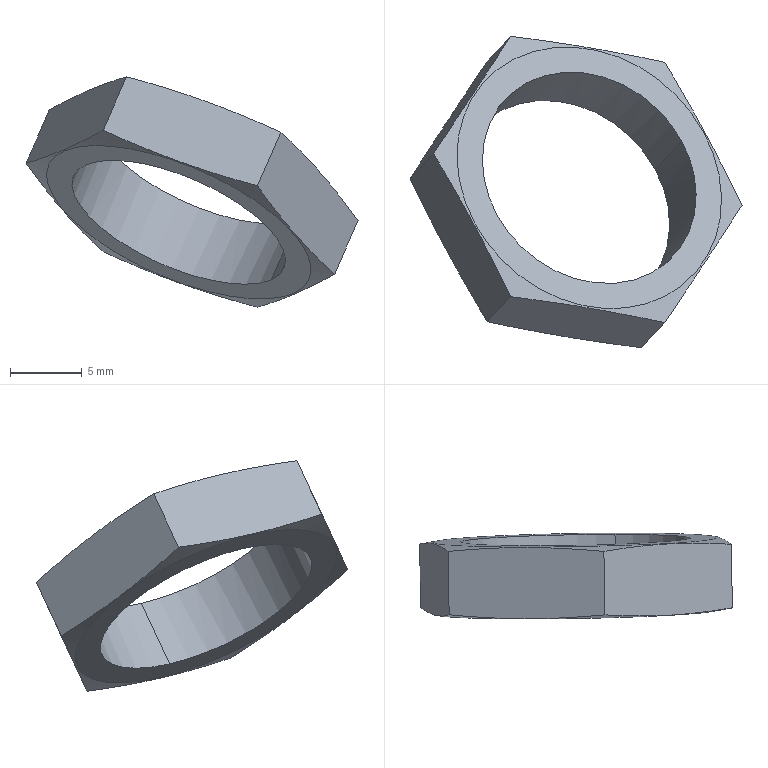Component | SolidWorks | 1369126_DSM_40_270_CC_HD_A_B_0-1_Flachmutter_M16x1_5_20-1 | 1 solid | 14 faces | box 23.1 x 21.66 x 16.04 mm | volume 720 mm3 | plane 8 | cone 4 | cylinder 2 | commonest cylinder face diameters 16 x2
STEP:
#1=COLOUR_RGB('',0.7922,0.8196,0.9333);
#2=FILL_AREA_STYLE_COLOUR('',#1);
#3=FILL_AREA_STYLE('',(#2));
#4=SURFACE_STYLE_FILL_AREA(#3);
#5=SURFACE_SIDE_STYLE('',(#4));
#6=SURFACE_STYLE_USAGE(.BOTH.,#5);
#7=PRESENTATION_STYLE_ASSIGNMENT((#6));
#8=CARTESIAN_POINT('',(-8.237,80.701,9.666));
#9=VERTEX_POINT('',#8);
#10=CARTESIAN_POINT('',(-7.73,80.902,9.351));
#11=VERTEX_POINT('',#10);
#12=CARTESIAN_POINT('',(-8.237,80.701,9.666));
#13=CARTESIAN_POINT('',(-8.246,80.719,9.662));
#14=CARTESIAN_POINT('',(-8.254,80.738,9.657));
#15=CARTESIAN_POINT('',(-8.267,80.775,9.645));
#16=CARTESIAN_POINT('',(-8.271,80.794,9.638));
#17=CARTESIAN_POINT('',(-8.276,80.832,9.622));
#18=CARTESIAN_POINT('',(-8.277,80.851,9.614));
#19=CARTESIAN_POINT('',(-8.274,80.888,9.596));
#20=CARTESIAN_POINT('',(-8.271,80.906,9.586));
#21=CARTESIAN_POINT('',(-8.261,80.94,9.565));
#22=CARTESIAN_POINT('',(-8.254,80.957,9.555));
#23=CARTESIAN_POINT('',(-8.237,80.987,9.533));
#24=CARTESIAN_POINT('',(-8.227,81.001,9.522));
#25=CARTESIAN_POINT('',(-8.204,81.027,9.5));
#26=CARTESIAN_POINT('',(-8.191,81.039,9.489));
#27=CARTESIAN_POINT('',(-8.162,81.059,9.467));
#28=CARTESIAN_POINT('',(-8.146,81.067,9.456));
#29=CARTESIAN_POINT('',(-8.113,81.08,9.435));
#30=CARTESIAN_POINT('',(-8.096,81.085,9.425));
#31=CARTESIAN_POINT('',(-8.059,81.091,9.407));
#32=CARTESIAN_POINT('',(-8.041,81.092,9.398));
#33=CARTESIAN_POINT('',(-8.002,81.09,9.382));
#34=CARTESIAN_POINT('',(-7.983,81.088,9.375));
#35=CARTESIAN_POINT('',(-7.945,81.079,9.362));
#36=CARTESIAN_POINT('',(-7.926,81.073,9.357));
#37=CARTESIAN_POINT('',(-7.889,81.057,9.348));
#38=CARTESIAN_POINT('',(-7.871,81.047,9.345));
#39=CARTESIAN_POINT('',(-7.837,81.025,9.34));
#40=CARTESIAN_POINT('',(-7.82,81.012,9.339));
#41=CARTESIAN_POINT('',(-7.79,80.984,9.338));
#42=CARTESIAN_POINT('',(-7.776,80.969,9.339));
#43=CARTESIAN_POINT('',(-7.751,80.937,9.343));
#44=CARTESIAN_POINT('',(-7.739,80.92,9.346));
#45=CARTESIAN_POINT('',(-7.73,80.902,9.351));
#46=B_SPLINE_CURVE_WITH_KNOTS('',3,(#12,#13,#14,#15,#16,#17,#18,#19,#20,#21,#22,#23,#24,#25,#26,#27,#28,#29,#30,#31,#32,#33,#34,#35,#36,#37,#38,#39,#40,#41,#42,#43,#44,#45),.UNSPECIFIED.,.F.,.F.,(4,2,2,2,2,2,2,2,2,2,2,2,2,2,2,2,4),(-0.,0.03125,0.0625,0.09375,0.125,0.1562,0.1875,0.2187,0.25,0.2813,0.3125,0.3438,0.375,0.4063,0.4375,0.4688,0.5),.UNSPECIFIED.);
#47=EDGE_CURVE('',#9,#11,#46,.T.);
#48=ORIENTED_EDGE('',*,*,#47,.F.);
#49=CARTESIAN_POINT('',(-8.309,80.624,9.5));
#50=VERTEX_POINT('',#49);
#51=CARTESIAN_POINT('',(-8.237,80.701,9.666));
#52=DIRECTION('',(-0.3689,-0.3928,-0.8424));
#53=VECTOR('',#52,39.37);
#54=LINE('',#51,#53);
#55=EDGE_CURVE('',#9,#50,#54,.T.);
#56=ORIENTED_EDGE('',*,*,#55,.T.);
#57=CARTESIAN_POINT('',(-7.802,80.824,9.185));
#58=VERTEX_POINT('',#57);
#59=CARTESIAN_POINT('',(-8.056,80.724,9.342));
#60=DIRECTION('',(-0.3689,-0.3928,-0.8424));
#61=DIRECTION('',(0.8049,0.3181,-0.5009));
#62=AXIS2_PLACEMENT_3D('',#59,#60,#61);
#63=CIRCLE('',#62,0.315);
#64=EDGE_CURVE('',#50,#58,#63,.T.);
#65=ORIENTED_EDGE('',*,*,#64,.T.);
#66=CARTESIAN_POINT('',(-7.73,80.902,9.351));
#67=DIRECTION('',(-0.3689,-0.3928,-0.8424));
#68=VECTOR('',#67,39.37);
#69=LINE('',#66,#68);
#70=EDGE_CURVE('',#11,#58,#69,.T.);
#71=ORIENTED_EDGE('',*,*,#70,.F.);
#72=EDGE_LOOP('',(#48,#56,#65,#71));
#73=FACE_OUTER_BOUND('',#72,.T.);
#74=CARTESIAN_POINT('',(-7.983,80.802,9.508));
#75=DIRECTION('',(-0.3689,-0.3928,-0.8424));
#76=DIRECTION('',(0.8049,0.3181,-0.5009));
#77=AXIS2_PLACEMENT_3D('',#74,#75,#76);
#78=CYLINDRICAL_SURFACE('',#77,0.315);
#79=ADVANCED_FACE('',(#73),#78,.F.);
#80=CARTESIAN_POINT('',(-8.37,80.6,9.538));
#81=VERTEX_POINT('',#80);
#82=CARTESIAN_POINT('',(-7.742,80.848,9.147));
#83=VERTEX_POINT('',#82);
#84=CARTESIAN_POINT('',(-8.056,80.724,9.342));
#85=DIRECTION('',(0.3689,0.3928,0.8424));
#86=DIRECTION('',(-0.8049,-0.3181,0.5009));
#87=AXIS2_PLACEMENT_3D('',#84,#85,#86);
#88=CIRCLE('',#87,0.3898);
#89=EDGE_CURVE('',#81,#83,#88,.T.);
#90=ORIENTED_EDGE('',*,*,#89,.T.);
#91=CARTESIAN_POINT('',(-7.739,80.85,9.146));
#92=VERTEX_POINT('',#91);
#93=CARTESIAN_POINT('',(-7.742,80.848,9.147));
#94=DIRECTION('',(0.8568,0.3815,-0.347));
#95=VECTOR('',#94,39.37);
#96=LINE('',#93,#95);
#97=EDGE_CURVE('',#83,#92,#96,.T.);
#98=ORIENTED_EDGE('',*,*,#97,.T.);
#99=CARTESIAN_POINT('',(-7.629,80.658,9.2));
#100=VERTEX_POINT('',#99);
#101=CARTESIAN_POINT('',(-7.739,80.85,9.146));
#102=CARTESIAN_POINT('',(-7.704,80.784,9.161));
#103=CARTESIAN_POINT('',(-7.667,80.721,9.179));
#104=CARTESIAN_POINT('',(-7.629,80.658,9.2));
#105=B_SPLINE_CURVE_WITH_KNOTS('',3,(#101,#102,#103,#104),.UNSPECIFIED.,.F.,.F.,(4,4),(0.01535,0.02114),.UNSPECIFIED.);
#106=EDGE_CURVE('',#92,#100,#105,.T.);
#107=ORIENTED_EDGE('',*,*,#106,.T.);
#108=CARTESIAN_POINT('',(-7.84,80.337,9.443));
#109=VERTEX_POINT('',#108);
#110=CARTESIAN_POINT('',(-7.629,80.658,9.2));
#111=CARTESIAN_POINT('',(-7.667,80.602,9.235));
#112=CARTESIAN_POINT('',(-7.74,80.491,9.309));
#113=CARTESIAN_POINT('',(-7.808,80.387,9.396));
#114=CARTESIAN_POINT('',(-7.84,80.337,9.443));
#115=B_SPLINE_CURVE_WITH_KNOTS('',3,(#110,#111,#112,#113,#114),.UNSPECIFIED.,.F.,.F.,(4,1,4),(0.00000023,0.005774,0.01155),.UNSPECIFIED.);
#116=EDGE_CURVE('',#100,#109,#115,.T.);
#117=ORIENTED_EDGE('',*,*,#116,.T.);
#118=CARTESIAN_POINT('',(-8.263,80.407,9.595));
#119=VERTEX_POINT('',#118);
#120=CARTESIAN_POINT('',(-7.84,80.337,9.443));
#121=CARTESIAN_POINT('',(-7.913,80.346,9.462));
#122=CARTESIAN_POINT('',(-8.057,80.366,9.506));
#123=CARTESIAN_POINT('',(-8.195,80.393,9.564));
#124=CARTESIAN_POINT('',(-8.263,80.407,9.595));
#125=B_SPLINE_CURVE_WITH_KNOTS('',3,(#120,#121,#122,#123,#124),.UNSPECIFIED.,.F.,.F.,(4,1,4),(0.00000023,0.005774,0.01155),.UNSPECIFIED.);
#126=EDGE_CURVE('',#109,#119,#125,.T.);
#127=ORIENTED_EDGE('',*,*,#126,.T.);
#128=CARTESIAN_POINT('',(-8.373,80.599,9.54));
#129=VERTEX_POINT('',#128);
#130=CARTESIAN_POINT('',(-8.263,80.407,9.595));
#131=CARTESIAN_POINT('',(-8.301,80.47,9.574));
#132=CARTESIAN_POINT('',(-8.337,80.534,9.555));
#133=CARTESIAN_POINT('',(-8.373,80.599,9.54));
#134=B_SPLINE_CURVE_WITH_KNOTS('',3,(#130,#131,#132,#133),.UNSPECIFIED.,.F.,.F.,(4,4),(0.02183,0.02762),.UNSPECIFIED.);
#135=EDGE_CURVE('',#119,#129,#134,.T.);
#136=ORIENTED_EDGE('',*,*,#135,.T.);
#137=CARTESIAN_POINT('',(-8.37,80.6,9.538));
#138=DIRECTION('',(-0.7286,-0.2451,0.6395));
#139=VECTOR('',#138,39.37);
#140=LINE('',#137,#139);
#141=EDGE_CURVE('',#81,#129,#140,.T.);
#142=ORIENTED_EDGE('',*,*,#141,.F.);
#143=EDGE_LOOP('',(#90,#98,#107,#117,#127,#136,#142));
#144=FACE_OUTER_BOUND('',#143,.T.);
#145=CARTESIAN_POINT('',(-8.056,80.724,9.342));
#146=DIRECTION('',(0.3689,0.3928,0.8424));
#147=DIRECTION('',(-0.8049,-0.3181,0.5009));
#148=AXIS2_PLACEMENT_3D('',#145,#146,#147);
#149=CONICAL_SURFACE('',#148,0.3898,1.396);
#150=ADVANCED_FACE('',(#144),#149,.T.);
#151=CARTESIAN_POINT('',(-8.297,80.678,9.704));
#152=VERTEX_POINT('',#151);
#153=CARTESIAN_POINT('',(-7.67,80.926,9.313));
#154=VERTEX_POINT('',#153);
#155=CARTESIAN_POINT('',(-7.983,80.802,9.508));
#156=DIRECTION('',(0.3689,0.3928,0.8424));
#157=DIRECTION('',(-0.8049,-0.3181,0.5009));
#158=AXIS2_PLACEMENT_3D('',#155,#156,#157);
#159=CIRCLE('',#158,0.3898);
#160=EDGE_CURVE('',#152,#154,#159,.T.);
#161=ORIENTED_EDGE('',*,*,#160,.F.);
#162=CARTESIAN_POINT('',(-8.3,80.676,9.705));
#163=VERTEX_POINT('',#162);
#164=CARTESIAN_POINT('',(-8.437,80.615,9.76));
#165=DIRECTION('',(-0.8568,-0.3815,0.347));
#166=VECTOR('',#165,39.37);
#167=LINE('',#164,#166);
#168=EDGE_CURVE('',#152,#163,#167,.T.);
#169=ORIENTED_EDGE('',*,*,#168,.T.);
#170=CARTESIAN_POINT('',(-8.199,80.476,9.741));
#171=VERTEX_POINT('',#170);
#172=CARTESIAN_POINT('',(-8.3,80.676,9.705));
#173=CARTESIAN_POINT('',(-8.265,80.611,9.72));
#174=CARTESIAN_POINT('',(-8.232,80.544,9.732));
#175=CARTESIAN_POINT('',(-8.199,80.476,9.741));
#176=B_SPLINE_CURVE_WITH_KNOTS('',3,(#172,#173,#174,#175),.UNSPECIFIED.,.F.,.F.,(4,4),(0.01535,0.02114),.UNSPECIFIED.);
#177=EDGE_CURVE('',#163,#171,#176,.T.);
#178=ORIENTED_EDGE('',*,*,#177,.T.);
#179=CARTESIAN_POINT('',(-7.776,80.405,9.589));
#180=VERTEX_POINT('',#179);
#181=CARTESIAN_POINT('',(-8.199,80.476,9.741));
#182=CARTESIAN_POINT('',(-8.126,80.467,9.721));
#183=CARTESIAN_POINT('',(-7.982,80.446,9.678));
#184=CARTESIAN_POINT('',(-7.844,80.419,9.62));
#185=CARTESIAN_POINT('',(-7.776,80.405,9.589));
#186=B_SPLINE_CURVE_WITH_KNOTS('',3,(#181,#182,#183,#184,#185),.UNSPECIFIED.,.F.,.F.,(4,1,4),(0.00000023,0.005774,0.01155),.UNSPECIFIED.);
#187=EDGE_CURVE('',#171,#180,#186,.T.);
#188=ORIENTED_EDGE('',*,*,#187,.T.);
#189=CARTESIAN_POINT('',(-7.565,80.726,9.347));
#190=VERTEX_POINT('',#189);
#191=CARTESIAN_POINT('',(-7.776,80.405,9.589));
#192=CARTESIAN_POINT('',(-7.739,80.461,9.554));
#193=CARTESIAN_POINT('',(-7.665,80.571,9.48));
#194=CARTESIAN_POINT('',(-7.598,80.675,9.393));
#195=CARTESIAN_POINT('',(-7.565,80.726,9.347));
#196=B_SPLINE_CURVE_WITH_KNOTS('',3,(#191,#192,#193,#194,#195),.UNSPECIFIED.,.F.,.F.,(4,1,4),(0.00000023,0.005774,0.01155),.UNSPECIFIED.);
#197=EDGE_CURVE('',#180,#190,#196,.T.);
#198=ORIENTED_EDGE('',*,*,#197,.T.);
#199=CARTESIAN_POINT('',(-7.667,80.927,9.311));
#200=VERTEX_POINT('',#199);
#201=CARTESIAN_POINT('',(-7.565,80.726,9.347));
#202=CARTESIAN_POINT('',(-7.598,80.794,9.337));
#203=CARTESIAN_POINT('',(-7.631,80.861,9.326));
#204=CARTESIAN_POINT('',(-7.667,80.927,9.311));
#205=B_SPLINE_CURVE_WITH_KNOTS('',3,(#201,#202,#203,#204),.UNSPECIFIED.,.F.,.F.,(4,4),(0.02183,0.02762),.UNSPECIFIED.);
#206=EDGE_CURVE('',#190,#200,#205,.T.);
#207=ORIENTED_EDGE('',*,*,#206,.T.);
#208=CARTESIAN_POINT('',(-7.55,80.966,9.208));
#209=DIRECTION('',(0.7286,0.2451,-0.6395));
#210=VECTOR('',#209,39.37);
#211=LINE('',#208,#210);
#212=EDGE_CURVE('',#154,#200,#211,.T.);
#213=ORIENTED_EDGE('',*,*,#212,.F.);
#214=EDGE_LOOP('',(#161,#169,#178,#188,#198,#207,#213));
#215=FACE_OUTER_BOUND('',#214,.T.);
#216=CARTESIAN_POINT('',(-7.994,80.79,9.484));
#217=DIRECTION('',(-0.3689,-0.3928,-0.8424));
#218=DIRECTION('',(0.8049,0.3181,-0.5009));
#219=AXIS2_PLACEMENT_3D('',#216,#217,#218);
#220=CONICAL_SURFACE('',#219,0.5512,1.396);
#221=ADVANCED_FACE('',(#215),#220,.T.);
#222=CARTESIAN_POINT('',(-7.73,80.902,9.351));
#223=CARTESIAN_POINT('',(-7.72,80.884,9.355));
#224=CARTESIAN_POINT('',(-7.712,80.866,9.36));
#225=CARTESIAN_POINT('',(-7.7,80.828,9.372));
#226=CARTESIAN_POINT('',(-7.696,80.809,9.379));
#227=CARTESIAN_POINT('',(-7.691,80.771,9.394));
#228=CARTESIAN_POINT('',(-7.69,80.752,9.403));
#229=CARTESIAN_POINT('',(-7.692,80.715,9.421));
#230=CARTESIAN_POINT('',(-7.696,80.698,9.431));
#231=CARTESIAN_POINT('',(-7.706,80.663,9.451));
#232=CARTESIAN_POINT('',(-7.712,80.647,9.462));
#233=CARTESIAN_POINT('',(-7.729,80.616,9.484));
#234=CARTESIAN_POINT('',(-7.739,80.602,9.495));
#235=CARTESIAN_POINT('',(-7.763,80.576,9.517));
#236=CARTESIAN_POINT('',(-7.776,80.565,9.528));
#237=CARTESIAN_POINT('',(-7.805,80.545,9.55));
#238=CARTESIAN_POINT('',(-7.82,80.536,9.561));
#239=CARTESIAN_POINT('',(-7.854,80.523,9.581));
#240=CARTESIAN_POINT('',(-7.871,80.518,9.591));
#241=CARTESIAN_POINT('',(-7.907,80.513,9.61));
#242=CARTESIAN_POINT('',(-7.926,80.511,9.619));
#243=CARTESIAN_POINT('',(-7.964,80.513,9.635));
#244=CARTESIAN_POINT('',(-7.983,80.516,9.642));
#245=CARTESIAN_POINT('',(-8.022,80.524,9.654));
#246=CARTESIAN_POINT('',(-8.041,80.531,9.66));
#247=CARTESIAN_POINT('',(-8.078,80.547,9.669));
#248=CARTESIAN_POINT('',(-8.096,80.556,9.672));
#249=CARTESIAN_POINT('',(-8.13,80.578,9.677));
#250=CARTESIAN_POINT('',(-8.146,80.591,9.678));
#251=CARTESIAN_POINT('',(-8.177,80.619,9.678));
#252=CARTESIAN_POINT('',(-8.191,80.634,9.677));
#253=CARTESIAN_POINT('',(-8.216,80.667,9.673));
#254=CARTESIAN_POINT('',(-8.227,80.684,9.67));
#255=CARTESIAN_POINT('',(-8.237,80.701,9.666));
#256=B_SPLINE_CURVE_WITH_KNOTS('',3,(#222,#223,#224,#225,#226,#227,#228,#229,#230,#231,#232,#233,#234,#235,#236,#237,#238,#239,#240,#241,#242,#243,#244,#245,#246,#247,#248,#249,#250,#251,#252,#253,#254,#255),.UNSPECIFIED.,.F.,.F.,(4,2,2,2,2,2,2,2,2,2,2,2,2,2,2,2,4),(0.5,0.5313,0.5625,0.5938,0.625,0.6563,0.6875,0.7188,0.75,0.7813,0.8125,0.8438,0.875,0.9063,0.9375,0.9688,1.),.UNSPECIFIED.);
#257=EDGE_CURVE('',#11,#9,#256,.T.);
#258=ORIENTED_EDGE('',*,*,#257,.T.);
#259=ORIENTED_EDGE('',*,*,#47,.T.);
#260=EDGE_LOOP('',(#258,#259));
#261=FACE_BOUND('',#260,.T.);
#262=CARTESIAN_POINT('',(-7.983,80.802,9.508));
#263=DIRECTION('',(0.3689,0.3928,0.8424));
#264=DIRECTION('',(-0.8049,-0.3181,0.5009));
#265=AXIS2_PLACEMENT_3D('',#262,#263,#264);
#266=CIRCLE('',#265,0.3898);
#267=EDGE_CURVE('',#154,#152,#266,.T.);
#268=ORIENTED_EDGE('',*,*,#267,.T.);
#269=ORIENTED_EDGE('',*,*,#160,.T.);
#270=EDGE_LOOP('',(#268,#269));
#271=FACE_OUTER_BOUND('',#270,.T.);
#272=CARTESIAN_POINT('',(-7.983,80.802,9.508));
#273=DIRECTION('',(-0.3689,-0.3928,-0.8424));
#274=DIRECTION('',(0.8049,0.3181,-0.5009));
#275=AXIS2_PLACEMENT_3D('',#272,#273,#274);
#276=PLANE('',#275);
#277=ADVANCED_FACE('',(#261,#271),#276,.F.);
#278=ORIENTED_EDGE('',*,*,#168,.F.);
#279=ORIENTED_EDGE('',*,*,#267,.F.);
#280=ORIENTED_EDGE('',*,*,#212,.T.);
#281=CARTESIAN_POINT('',(-7.776,81.118,9.256));
#282=VERTEX_POINT('',#281);
#283=CARTESIAN_POINT('',(-7.667,80.927,9.311));
#284=CARTESIAN_POINT('',(-7.684,80.959,9.303));
#285=CARTESIAN_POINT('',(-7.702,80.992,9.295));
#286=CARTESIAN_POINT('',(-7.739,81.055,9.276));
#287=CARTESIAN_POINT('',(-7.757,81.087,9.267));
#288=CARTESIAN_POINT('',(-7.776,81.118,9.256));
#289=B_SPLINE_CURVE_WITH_KNOTS('',3,(#283,#284,#285,#286,#287,#288),.UNSPECIFIED.,.F.,.F.,(4,2,4),(0.02762,0.03051,0.03341),.UNSPECIFIED.);
#290=EDGE_CURVE('',#200,#282,#289,.T.);
#291=ORIENTED_EDGE('',*,*,#290,.T.);
#292=CARTESIAN_POINT('',(-8.199,81.189,9.408));
#293=VERTEX_POINT('',#292);
#294=CARTESIAN_POINT('',(-7.776,81.118,9.256));
#295=CARTESIAN_POINT('',(-7.844,81.133,9.287));
#296=CARTESIAN_POINT('',(-7.982,81.16,9.345));
#297=CARTESIAN_POINT('',(-8.126,81.18,9.389));
#298=CARTESIAN_POINT('',(-8.199,81.189,9.408));
#299=B_SPLINE_CURVE_WITH_KNOTS('',3,(#294,#295,#296,#297,#298),.UNSPECIFIED.,.F.,.F.,(4,1,4),(0.00000023,0.005774,0.01155),.UNSPECIFIED.);
#300=EDGE_CURVE('',#282,#293,#299,.T.);
#301=ORIENTED_EDGE('',*,*,#300,.T.);
#302=CARTESIAN_POINT('',(-8.41,80.868,9.651));
#303=VERTEX_POINT('',#302);
#304=CARTESIAN_POINT('',(-8.199,81.189,9.408));
#305=CARTESIAN_POINT('',(-8.232,81.138,9.454));
#306=CARTESIAN_POINT('',(-8.299,81.034,9.542));
#307=CARTESIAN_POINT('',(-8.372,80.924,9.616));
#308=CARTESIAN_POINT('',(-8.41,80.868,9.651));
#309=B_SPLINE_CURVE_WITH_KNOTS('',3,(#304,#305,#306,#307,#308),.UNSPECIFIED.,.F.,.F.,(4,1,4),(0.00000023,0.005774,0.01155),.UNSPECIFIED.);
#310=EDGE_CURVE('',#293,#303,#309,.T.);
#311=ORIENTED_EDGE('',*,*,#310,.T.);
#312=CARTESIAN_POINT('',(-8.41,80.868,9.651));
#313=CARTESIAN_POINT('',(-8.391,80.837,9.661));
#314=CARTESIAN_POINT('',(-8.373,80.805,9.671));
#315=CARTESIAN_POINT('',(-8.336,80.741,9.689));
#316=CARTESIAN_POINT('',(-8.318,80.709,9.697));
#317=CARTESIAN_POINT('',(-8.3,80.676,9.705));
#318=B_SPLINE_CURVE_WITH_KNOTS('',3,(#312,#313,#314,#315,#316,#317),.UNSPECIFIED.,.F.,.F.,(4,2,4),(0.009565,0.01246,0.01535),.UNSPECIFIED.);
#319=EDGE_CURVE('',#303,#163,#318,.T.);
#320=ORIENTED_EDGE('',*,*,#319,.T.);
#321=EDGE_LOOP('',(#278,#279,#280,#291,#301,#311,#320));
#322=FACE_OUTER_BOUND('',#321,.T.);
#323=CARTESIAN_POINT('',(-7.994,80.79,9.484));
#324=DIRECTION('',(-0.3689,-0.3928,-0.8424));
#325=DIRECTION('',(0.8049,0.3181,-0.5009));
#326=AXIS2_PLACEMENT_3D('',#323,#324,#325);
#327=CONICAL_SURFACE('',#326,0.5512,1.396);
#328=ADVANCED_FACE('',(#322),#327,.T.);
#329=ORIENTED_EDGE('',*,*,#97,.F.);
#330=CARTESIAN_POINT('',(-8.056,80.724,9.342));
#331=DIRECTION('',(0.3689,0.3928,0.8424));
#332=DIRECTION('',(-0.8049,-0.3181,0.5009));
#333=AXIS2_PLACEMENT_3D('',#330,#331,#332);
#334=CIRCLE('',#333,0.3898);
#335=EDGE_CURVE('',#83,#81,#334,.T.);
#336=ORIENTED_EDGE('',*,*,#335,.T.);
#337=ORIENTED_EDGE('',*,*,#141,.T.);
#338=CARTESIAN_POINT('',(-8.474,80.8,9.504));
#339=VERTEX_POINT('',#338);
#340=CARTESIAN_POINT('',(-8.373,80.599,9.54));
#341=CARTESIAN_POINT('',(-8.39,80.632,9.533));
#342=CARTESIAN_POINT('',(-8.407,80.665,9.526));
#343=CARTESIAN_POINT('',(-8.441,80.732,9.514));
#344=CARTESIAN_POINT('',(-8.458,80.766,9.509));
#345=CARTESIAN_POINT('',(-8.474,80.8,9.504));
#346=B_SPLINE_CURVE_WITH_KNOTS('',3,(#340,#341,#342,#343,#344,#345),.UNSPECIFIED.,.F.,.F.,(4,2,4),(0.02762,0.03051,0.03341),.UNSPECIFIED.);
#347=EDGE_CURVE('',#129,#339,#346,.T.);
#348=ORIENTED_EDGE('',*,*,#347,.T.);
#349=CARTESIAN_POINT('',(-8.263,81.121,9.262));
#350=VERTEX_POINT('',#349);
#351=CARTESIAN_POINT('',(-8.474,80.8,9.504));
#352=CARTESIAN_POINT('',(-8.442,80.851,9.458));
#353=CARTESIAN_POINT('',(-8.374,80.955,9.37));
#354=CARTESIAN_POINT('',(-8.301,81.065,9.297));
#355=CARTESIAN_POINT('',(-8.263,81.121,9.262));
#356=B_SPLINE_CURVE_WITH_KNOTS('',3,(#351,#352,#353,#354,#355),.UNSPECIFIED.,.F.,.F.,(4,1,4),(0.00000023,0.005774,0.01155),.UNSPECIFIED.);
#357=EDGE_CURVE('',#339,#350,#356,.T.);
#358=ORIENTED_EDGE('',*,*,#357,.T.);
#359=CARTESIAN_POINT('',(-7.84,81.05,9.11));
#360=VERTEX_POINT('',#359);
#361=CARTESIAN_POINT('',(-8.263,81.121,9.262));
#362=CARTESIAN_POINT('',(-8.195,81.107,9.231));
#363=CARTESIAN_POINT('',(-8.057,81.08,9.173));
#364=CARTESIAN_POINT('',(-7.913,81.059,9.129));
#365=CARTESIAN_POINT('',(-7.84,81.05,9.11));
#366=B_SPLINE_CURVE_WITH_KNOTS('',3,(#361,#362,#363,#364,#365),.UNSPECIFIED.,.F.,.F.,(4,1,4),(0.00000023,0.005774,0.01155),.UNSPECIFIED.);
#367=EDGE_CURVE('',#350,#360,#366,.T.);
#368=ORIENTED_EDGE('',*,*,#367,.T.);
#369=CARTESIAN_POINT('',(-7.84,81.05,9.11));
#370=CARTESIAN_POINT('',(-7.824,81.016,9.114));
#371=CARTESIAN_POINT('',(-7.807,80.982,9.12));
#372=CARTESIAN_POINT('',(-7.774,80.916,9.132));
#373=CARTESIAN_POINT('',(-7.756,80.882,9.138));
#374=CARTESIAN_POINT('',(-7.739,80.85,9.146));
#375=B_SPLINE_CURVE_WITH_KNOTS('',3,(#369,#370,#371,#372,#373,#374),.UNSPECIFIED.,.F.,.F.,(4,2,4),(0.009565,0.01246,0.01535),.UNSPECIFIED.);
#376=EDGE_CURVE('',#360,#92,#375,.T.);
#377=ORIENTED_EDGE('',*,*,#376,.T.);
#378=EDGE_LOOP('',(#329,#336,#337,#348,#358,#368,#377));
#379=FACE_OUTER_BOUND('',#378,.T.);
#380=CARTESIAN_POINT('',(-8.056,80.724,9.342));
#381=DIRECTION('',(0.3689,0.3928,0.8424));
#382=DIRECTION('',(-0.8049,-0.3181,0.5009));
#383=AXIS2_PLACEMENT_3D('',#380,#381,#382);
#384=CONICAL_SURFACE('',#383,0.3898,1.396);
#385=ADVANCED_FACE('',(#379),#384,.T.);
#386=CARTESIAN_POINT('',(-8.056,80.724,9.342));
#387=DIRECTION('',(-0.3689,-0.3928,-0.8424));
#388=DIRECTION('',(0.8049,0.3181,-0.5009));
#389=AXIS2_PLACEMENT_3D('',#386,#387,#388);
#390=CIRCLE('',#389,0.315);
#391=EDGE_CURVE('',#58,#50,#390,.T.);
#392=ORIENTED_EDGE('',*,*,#391,.F.);
#393=ORIENTED_EDGE('',*,*,#64,.F.);
#394=EDGE_LOOP('',(#392,#393));
#395=FACE_BOUND('',#394,.T.);
#396=ORIENTED_EDGE('',*,*,#89,.F.);
#397=ORIENTED_EDGE('',*,*,#335,.F.);
#398=EDGE_LOOP('',(#396,#397));
#399=FACE_OUTER_BOUND('',#398,.T.);
#400=CARTESIAN_POINT('',(-7.875,80.388,9.42));
#401=DIRECTION('',(0.3689,0.3928,0.8424));
#402=DIRECTION('',(-0.8049,-0.3181,0.5009));
#403=AXIS2_PLACEMENT_3D('',#400,#401,#402);
#404=PLANE('',#403);
#405=ADVANCED_FACE('',(#395,#399),#404,.F.);
#406=CARTESIAN_POINT('',(-8.267,80.403,9.585));
#407=DIRECTION('',(0.3689,0.3928,0.8424));
#408=VECTOR('',#407,39.37);
#409=LINE('',#406,#408);
#410=EDGE_CURVE('',#119,#171,#409,.T.);
#411=ORIENTED_EDGE('',*,*,#410,.F.);
#412=ORIENTED_EDGE('',*,*,#126,.F.);
#413=CARTESIAN_POINT('',(-7.845,80.332,9.433));
#414=DIRECTION('',(0.3689,0.3928,0.8424));
#415=VECTOR('',#414,39.37);
#416=LINE('',#413,#415);
#417=EDGE_CURVE('',#109,#180,#416,.T.);
#418=ORIENTED_EDGE('',*,*,#417,.T.);
#419=ORIENTED_EDGE('',*,*,#187,.F.);
#420=EDGE_LOOP('',(#411,#412,#418,#419));
#421=FACE_OUTER_BOUND('',#420,.T.);
#422=CARTESIAN_POINT('',(-7.845,80.332,9.433));
#423=DIRECTION('',(-0.,0.9063,-0.4226));
#424=DIRECTION('',(0.9295,-0.1559,-0.3344));
#425=AXIS2_PLACEMENT_3D('',#422,#423,#424);
#426=PLANE('',#425);
#427=ADVANCED_FACE('',(#421),#426,.F.);
#428=CARTESIAN_POINT('',(-8.478,80.795,9.495));
#429=DIRECTION('',(0.3689,0.3928,0.8424));
#430=VECTOR('',#429,39.37);
#431=LINE('',#428,#430);
#432=EDGE_CURVE('',#339,#303,#431,.T.);
#433=ORIENTED_EDGE('',*,*,#432,.F.);
#434=ORIENTED_EDGE('',*,*,#347,.F.);
#435=ORIENTED_EDGE('',*,*,#135,.F.);
#436=ORIENTED_EDGE('',*,*,#410,.T.);
#437=ORIENTED_EDGE('',*,*,#177,.F.);
#438=ORIENTED_EDGE('',*,*,#319,.F.);
#439=EDGE_LOOP('',(#433,#434,#435,#436,#437,#438));
#440=FACE_OUTER_BOUND('',#439,.T.);
#441=CARTESIAN_POINT('',(-8.267,80.403,9.585));
#442=DIRECTION('',(0.8049,0.3181,-0.5009));
#443=DIRECTION('',(0.3689,0.3928,0.8424));
#444=AXIS2_PLACEMENT_3D('',#441,#442,#443);
#445=PLANE('',#444);
#446=ADVANCED_FACE('',(#440),#445,.F.);
#447=CARTESIAN_POINT('',(-8.267,81.117,9.252));
#448=DIRECTION('',(0.3689,0.3928,0.8424));
#449=VECTOR('',#448,39.37);
#450=LINE('',#447,#449);
#451=EDGE_CURVE('',#350,#293,#450,.T.);
#452=ORIENTED_EDGE('',*,*,#451,.F.);
#453=ORIENTED_EDGE('',*,*,#357,.F.);
#454=ORIENTED_EDGE('',*,*,#432,.T.);
#455=ORIENTED_EDGE('',*,*,#310,.F.);
#456=EDGE_LOOP('',(#452,#453,#454,#455));
#457=FACE_OUTER_BOUND('',#456,.T.);
#458=CARTESIAN_POINT('',(-8.478,80.795,9.495));
#459=DIRECTION('',(0.8049,-0.5882,-0.07826));
#460=DIRECTION('',(-0.4647,-0.7069,0.5332));
#461=AXIS2_PLACEMENT_3D('',#458,#459,#460);
#462=PLANE('',#461);
#463=ADVANCED_FACE('',(#457),#462,.F.);
#464=CARTESIAN_POINT('',(-7.845,81.046,9.1));
#465=DIRECTION('',(0.3689,0.3928,0.8424));
#466=VECTOR('',#465,39.37);
#467=LINE('',#464,#466);
#468=EDGE_CURVE('',#360,#282,#467,.T.);
#469=ORIENTED_EDGE('',*,*,#468,.F.);
#470=ORIENTED_EDGE('',*,*,#367,.F.);
#471=ORIENTED_EDGE('',*,*,#451,.T.);
#472=ORIENTED_EDGE('',*,*,#300,.F.);
#473=EDGE_LOOP('',(#469,#470,#471,#472));
#474=FACE_OUTER_BOUND('',#473,.T.);
#475=CARTESIAN_POINT('',(-8.267,81.117,9.252));
#476=DIRECTION('',(0.,-0.9063,0.4226));
#477=DIRECTION('',(-0.9295,0.1559,0.3344));
#478=AXIS2_PLACEMENT_3D('',#475,#476,#477);
#479=PLANE('',#478);
#480=ADVANCED_FACE('',(#474),#479,.F.);
#481=CARTESIAN_POINT('',(-7.633,80.653,9.19));
#482=DIRECTION('',(0.3689,0.3928,0.8424));
#483=VECTOR('',#482,39.37);
#484=LINE('',#481,#483);
#485=EDGE_CURVE('',#100,#190,#484,.T.);
#486=ORIENTED_EDGE('',*,*,#485,.F.);
#487=ORIENTED_EDGE('',*,*,#106,.F.);
#488=ORIENTED_EDGE('',*,*,#376,.F.);
#489=ORIENTED_EDGE('',*,*,#468,.T.);
#490=ORIENTED_EDGE('',*,*,#290,.F.);
#491=ORIENTED_EDGE('',*,*,#206,.F.);
#492=EDGE_LOOP('',(#486,#487,#488,#489,#490,#491));
#493=FACE_OUTER_BOUND('',#492,.T.);
#494=CARTESIAN_POINT('',(-7.845,81.046,9.1));
#495=DIRECTION('',(-0.8049,-0.3181,0.5009));
#496=DIRECTION('',(-0.3689,-0.3928,-0.8424));
#497=AXIS2_PLACEMENT_3D('',#494,#495,#496);
#498=PLANE('',#497);
#499=ADVANCED_FACE('',(#493),#498,.F.);
#500=ORIENTED_EDGE('',*,*,#417,.F.);
#501=ORIENTED_EDGE('',*,*,#116,.F.);
#502=ORIENTED_EDGE('',*,*,#485,.T.);
#503=ORIENTED_EDGE('',*,*,#197,.F.);
#504=EDGE_LOOP('',(#500,#501,#502,#503));
#505=FACE_OUTER_BOUND('',#504,.T.);
#506=CARTESIAN_POINT('',(-7.633,80.653,9.19));
#507=DIRECTION('',(-0.8049,0.5882,0.07826));
#508=DIRECTION('',(0.4647,0.7069,-0.5332));
#509=AXIS2_PLACEMENT_3D('',#506,#507,#508);
#510=PLANE('',#509);
#511=ADVANCED_FACE('',(#505),#510,.F.);
#512=ORIENTED_EDGE('',*,*,#55,.F.);
#513=ORIENTED_EDGE('',*,*,#257,.F.);
#514=ORIENTED_EDGE('',*,*,#70,.T.);
#515=ORIENTED_EDGE('',*,*,#391,.T.);
#516=EDGE_LOOP('',(#512,#513,#514,#515));
#517=FACE_OUTER_BOUND('',#516,.T.);
#518=CARTESIAN_POINT('',(-7.983,80.802,9.508));
#519=DIRECTION('',(-0.3689,-0.3928,-0.8424));
#520=DIRECTION('',(0.8049,0.3181,-0.5009));
#521=AXIS2_PLACEMENT_3D('',#518,#519,#520);
#522=CYLINDRICAL_SURFACE('',#521,0.315);
#523=ADVANCED_FACE('',(#517),#522,.F.);
#524=CLOSED_SHELL('',(#79,#150,#221,#277,#328,#385,#405,#427,#446,#463,#480,#499,#511,#523));
#525=MANIFOLD_SOLID_BREP('',#524);
#526=STYLED_ITEM('',(#7),#525);
#527=PRESENTATION_LAYER_ASSIGNMENT('','',(#526));
#528=CARTESIAN_POINT('',(0.,0.,0.));
#529=DIRECTION('',(0.,0.,1.));
#530=DIRECTION('',(1.,0.,0.));
#531=AXIS2_PLACEMENT_3D('',#528,#529,#530);
#532=(LENGTH_UNIT()NAMED_UNIT(*)SI_UNIT($,.METRE.));
#533=LENGTH_MEASURE_WITH_UNIT(LENGTH_MEASURE(0.0254),#532);
#534=DIMENSIONAL_EXPONENTS(1.,0.,0.,0.,0.,0.,0.);
#535=(CONVERSION_BASED_UNIT('',#533)LENGTH_UNIT()NAMED_UNIT(#534));
#536=UNCERTAINTY_MEASURE_WITH_UNIT(LENGTH_MEASURE(0.00001),#535,'','');
#537=(NAMED_UNIT(*)PLANE_ANGLE_UNIT()SI_UNIT($,.RADIAN.));
#538=(NAMED_UNIT(*)SI_UNIT($,.STERADIAN.)SOLID_ANGLE_UNIT());
#539=(GEOMETRIC_REPRESENTATION_CONTEXT(3)GLOBAL_UNCERTAINTY_ASSIGNED_CONTEXT((#536))GLOBAL_UNIT_ASSIGNED_CONTEXT((#535,#537,#538))REPRESENTATION_CONTEXT('',''));
#540=ADVANCED_BREP_SHAPE_REPRESENTATION('',(#525,#531),#539);
#541=(LENGTH_UNIT()NAMED_UNIT(*)SI_UNIT($,.METRE.));
#542=LENGTH_MEASURE_WITH_UNIT(LENGTH_MEASURE(0.0254),#541);
#543=DIMENSIONAL_EXPONENTS(1.,0.,0.,0.,0.,0.,0.);
#544=(CONVERSION_BASED_UNIT('',#542)LENGTH_UNIT()NAMED_UNIT(#543));
#545=UNCERTAINTY_MEASURE_WITH_UNIT(LENGTH_MEASURE(0.00001),#544,'','');
#546=(NAMED_UNIT(*)PLANE_ANGLE_UNIT()SI_UNIT($,.RADIAN.));
#547=(NAMED_UNIT(*)SI_UNIT($,.STERADIAN.)SOLID_ANGLE_UNIT());
#548=(GEOMETRIC_REPRESENTATION_CONTEXT(3)GLOBAL_UNCERTAINTY_ASSIGNED_CONTEXT((#545))GLOBAL_UNIT_ASSIGNED_CONTEXT((#544,#546,#547))REPRESENTATION_CONTEXT('',''));
#549=MECHANICAL_DESIGN_GEOMETRIC_PRESENTATION_REPRESENTATION('',(#526),#548);